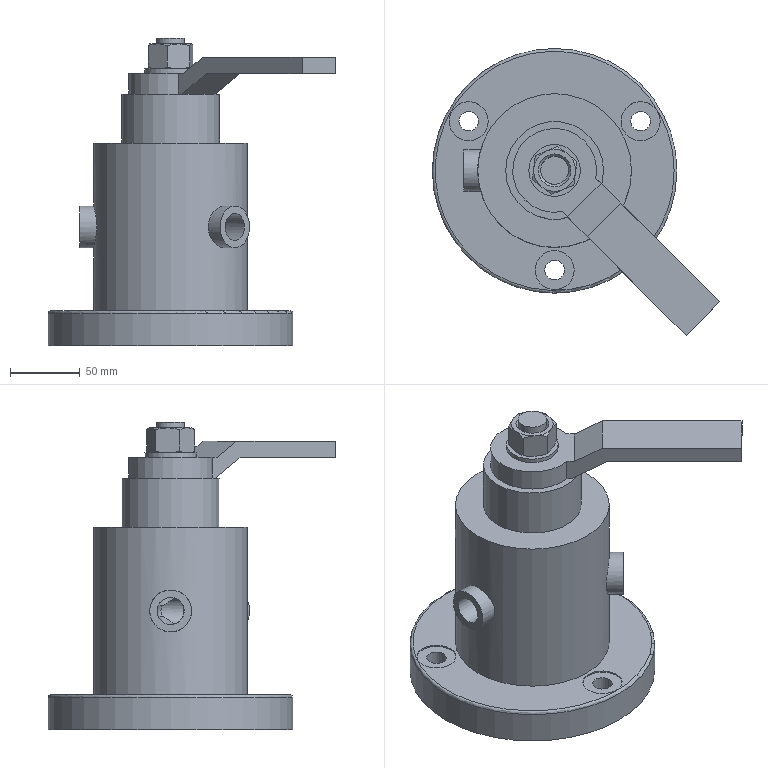Assembly | NX | mm | 7 component files | 7 solids | 100 faces | box 205.59 x 205.59 x 220 mm | volume 1937702 mm3 | plane 50 | cylinder 29 | cone 19 | torus 1 | sphere 1 | commonest cylinder face diameters 30 x4 19.5 x4 18 x3 60 x3 14 x3 28 x3 20 x2 5 x2
Bill of materials:
unnamed part 1 | 1 |  | Plain solid short cylinder (disc); diameter roughly 2.4 times its height.
GB-T97_1-2002,M20 | 1 |  | Flat, thin annular disc (plain ring/washer-like shape): a circular plate with one concentric circular through-hole, flat parallel faces, and straight cylindrical inner and outer edges.
unnamed part 2 | 1 |  | Flanged, stepped cylindrical hub: a round base flange, a larger cylindrical body, and a smaller top boss, with a central axial through-bore. There are three small holes on the flange and two small radial bosses with holes on the side of the body.
unnamed part 3 | 1 |  | Flat lever or strap of constant thickness. One end is a round eye with a square through-hole, and a straight rectangular arm comes off it. The arm has a joggle (offset bend) so the eye and the arm sit in parallel planes.
unnamed part 4 | 1 |  | Plain solid cylinder (slug or pin blank); diameter slightly larger than its length.
GB-T6170_F-2000,M20x2.5 | 1 |  | Hexagonal nut-like body with a central round through-bore, chamfered corners on both ends, and a chamfer or countersink at the bore entry.
unnamed part 5 | 1 |  | Stepped, coaxial shaft-like part: a tapered (conical) lower body, a narrower cylindrical middle shank, a short slightly wider band near the top (possibly a hex or flats with chamfer cuts), and a small cylindrical pin at the top. A transverse hole crosses the tapered body.
Mates:
1. fix | valve_seat 1 component
2. touch align | valve_core 1 face | valve_seat 1 face
3. concentric | valve_core 1 edge | valve_seat 1 edge
4. concentric | screw_plug 1 edge | valve_seat 1 edge
5. concentric | plug 1 edge | screw_plug 1 edge
6. center | wrench 1 face | wrench 1 face | valve_core 1 face | valve_core 1 face
7. center | wrench 1 face | wrench 1 face | valve_core 1 face | valve_core 1 face
8. touch align | wrench 1 face | valve_seat 1 face
9. touch align | wrench 1 face | valve_seat 1 face
10. concentric | washer 1 edge | valve_core 1 edge
11. concentric | nut 1 edge | washer 1 edge